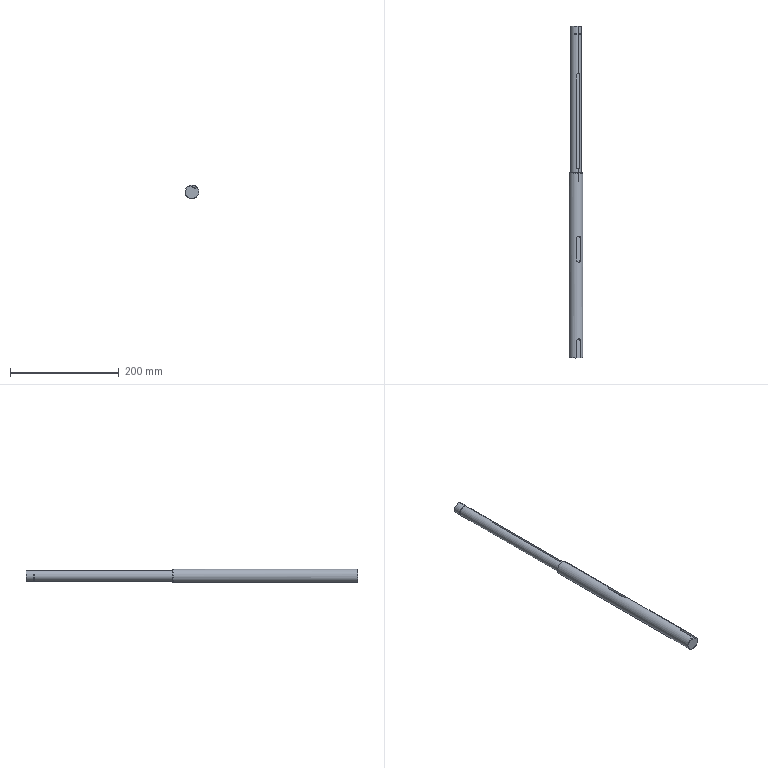Component | SolidWorks | -PullerDriveShaft-1 | 1 solid | 34 faces | box 25 x 610 x 25 mm | volume 245713 mm3 | cylinder 15 | plane 14 | cone 5 | commonest cylinder face diameters 8 x4 20 x4 6 x3 25 x2 19 x2
build123d program:
from build123d import *

# Parameters (mm, degrees)
CHAMFER1_SIZE      = 0.3
SKETCH9_W          = 2.5
SKETCH9_H          = 440
CHAMFER2_SIZE      = 0.5
CUT_EXTRUDE1_DEPTH = 3.5
CUT_EXTRUDE2_DEPTH = 4
SKETCH12_R         = 12.5
SKETCH12_R_2       = 10
CUT_EXTRUDE3_DEPTH = 100
CUT_EXTRUDE4_DEPTH = 4
CHAMFER3_SIZE      = 0.5


with BuildPart() as part:
    # Sketch1 → Revolve1 (revolve)
    with BuildSketch(Plane.XY):
        Polygon((0, 0), (10, 0), (10, 595), (9.5, 595), (9.5, 596.2), (10, 596.2), (10, 610), (0, 610), align=None)
    revolve(axis=Axis((0, -4012.913, 0), (0, 1, 0)))

    # Chamfer1
    chamfer1_edges = [part.edges().sort_by_distance(p)[0] for p in [
        (-10, 610, 0),
    ]]
    chamfer(chamfer1_edges, length=CHAMFER1_SIZE)

    # Sketch9 → Revolve2 (revolve)
    with BuildSketch(Plane.XY, mode=Mode.PRIVATE) as revolve2_sk:
        with Locations((11.25, 220)):
            Rectangle(SKETCH9_W, SKETCH9_H)
    revolve(revolve2_sk.sketch.rotate(Axis((0, -4012.913, 0), (0, -1, 0)), 180), axis=Axis((0, -4012.913, 0), (0, -1, 0)))

    # Chamfer2
    chamfer2_edges = [part.edges().sort_by_distance(p)[0] for p in [
        (12.5, 0, 0),
    ]]
    chamfer(chamfer2_edges, length=CHAMFER2_SIZE)

    # Sketch10 → Cut-Extrude1 (cut)
    with BuildSketch(Plane.ZY.offset(10)):
        with BuildLine():
            Line((3, 520), (3, 350))
            ThreePointArc((3, 350), (0, 347), (-3, 350))
            Line((-3, 350), (-3, 520))
            ThreePointArc((-3, 520), (0, 523), (3, 520))
        make_face()
    extrude(amount=-CUT_EXTRUDE1_DEPTH, mode=Mode.SUBTRACT)

    # Sketch11 → Cut-Extrude2 (cut)
    with BuildSketch(Plane.ZY.offset(12.5)):
        with BuildLine():
            Line((4, 220), (4, 180))
            ThreePointArc((4, 180), (0, 176), (-4, 180))
            Line((-4, 180), (-4, 220))
            ThreePointArc((-4, 220), (0, 224), (4, 220))
        make_face()
    extrude(amount=-CUT_EXTRUDE2_DEPTH, mode=Mode.SUBTRACT)

    # Sketch12 → Cut-Extrude3 (cut)
    with BuildSketch(Plane(origin=(0, 440, 0), x_dir=(1, 0, 0), z_dir=(0, 1, 0))):
        with Locations(Location((0, 0, 0), (0, 0, 180))):
            Circle(SKETCH12_R)
        Circle(SKETCH12_R_2, mode=Mode.SUBTRACT)
    extrude(amount=-CUT_EXTRUDE3_DEPTH, mode=Mode.SUBTRACT)

    # Sketch13 → Cut-Extrude4 (cut)
    with BuildSketch(Plane.ZY.offset(12.5)):
        with BuildLine():
            Line((4, 31), (4, -7.474))
            ThreePointArc((4, -7.474), (0, -11.474), (-4, -7.474))
            Line((-4, -7.474), (-4, 31))
            ThreePointArc((-4, 31), (0, 35), (4, 31))
        make_face()
    extrude(amount=-CUT_EXTRUDE4_DEPTH, mode=Mode.SUBTRACT)

    # Chamfer3
    chamfer3_edges = [part.edges().sort_by_distance(p)[0] for p in [
        (12.5, 340, 0),
    ]]
    chamfer(chamfer3_edges, length=CHAMFER3_SIZE)


solid = part.part

# Placed as in the assembly
solid = solid.moved(Location((205, 870, -173), (180, 66.949, -180)))